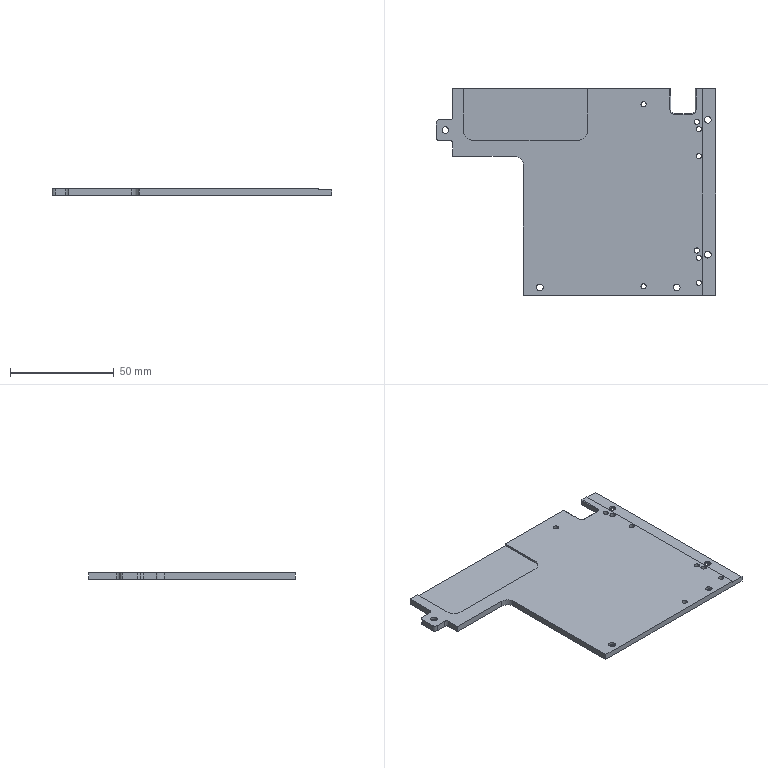CAM job | Mastercam | mm | 16 operations | part box 134.7 x 99.55 x 3
1. Contour (Ramp) | 8 - 8C
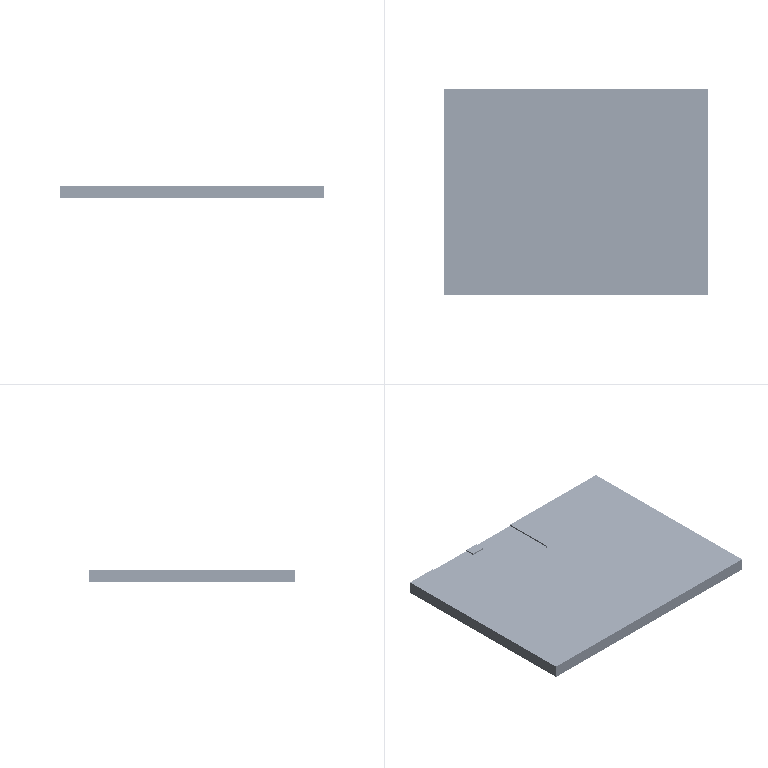2. Contour (Ramp) | 8 - 8C
3. Contour (2D) | 9 - 8J
4. Contour (2D) | 9 - 8J
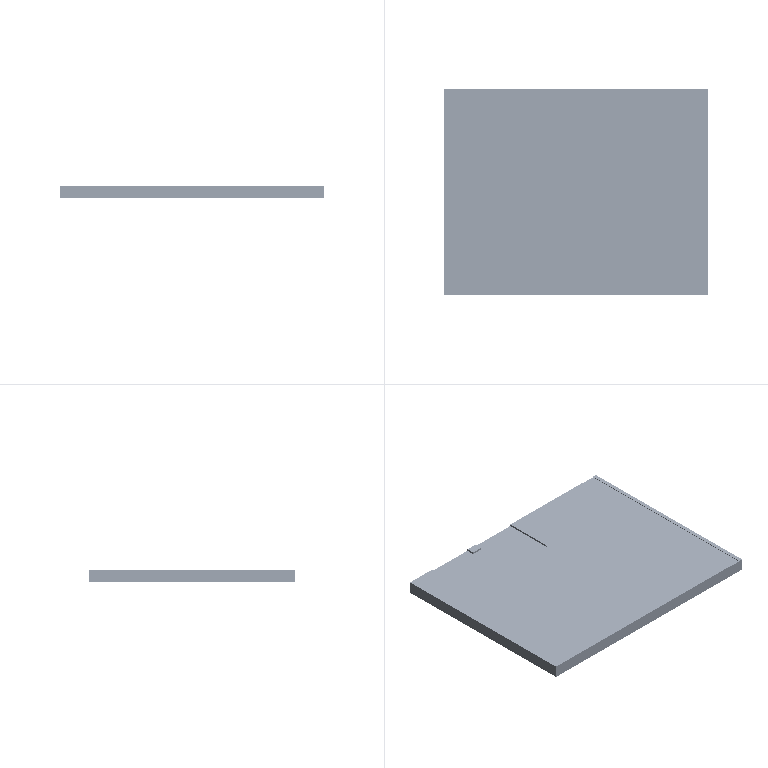5. Contour (2D) | 9 - 8J
6. Drill/Counterbore | 1 - 6 倒角刀
7. Drill/Counterbore | 1 - 6 倒角刀
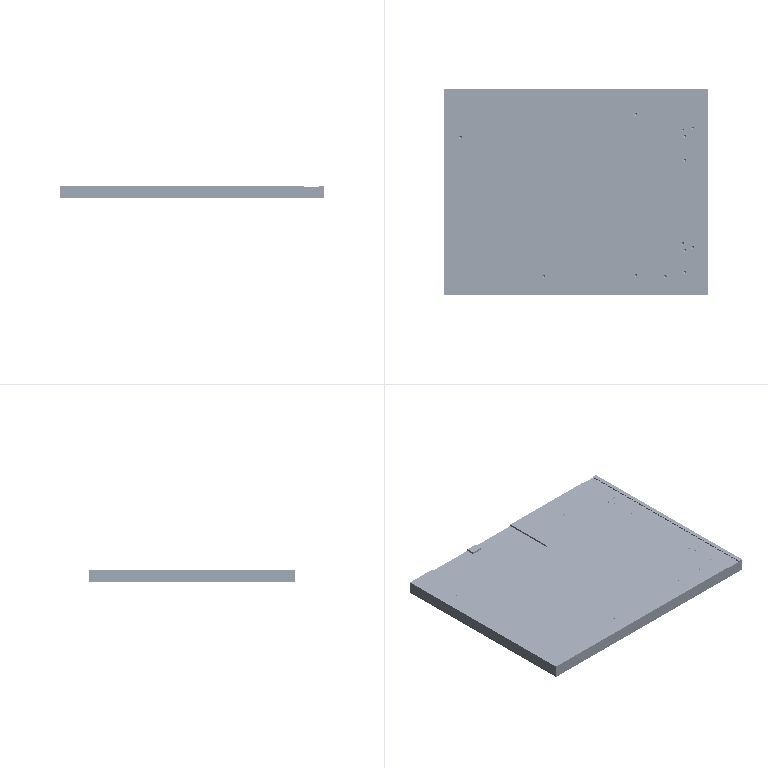8. Peck Drill | 21 - 3.2 钻头
9. Peck Drill | 14 - 2.5 钻头
10. Contour (Ramp) | 8 - 8C
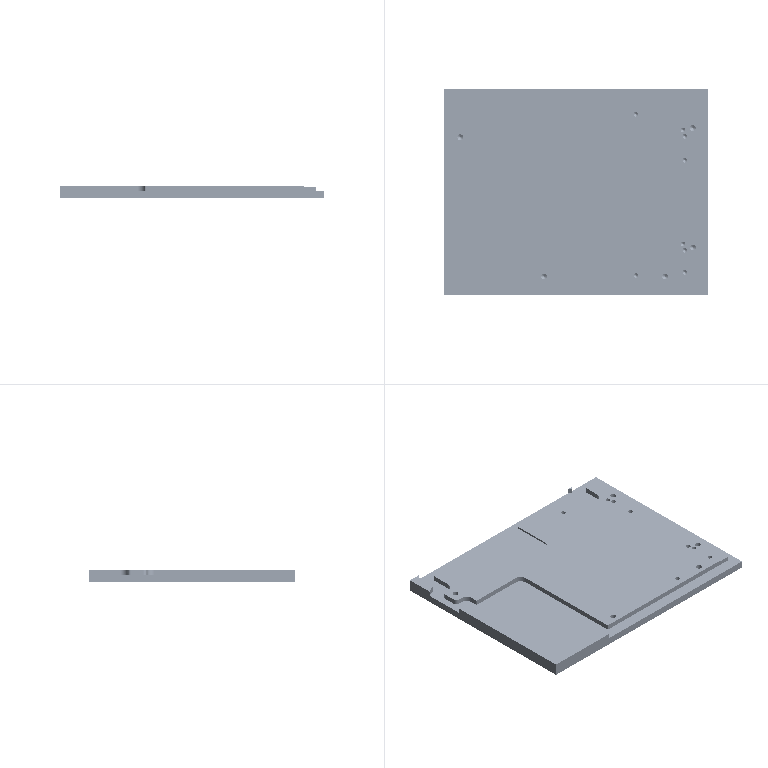11. Contour (2D) | 9 - 8J
12. Contour (Remachining) | 13 - 3J
13. Chamfer Drill | 1 - 6 倒角刀
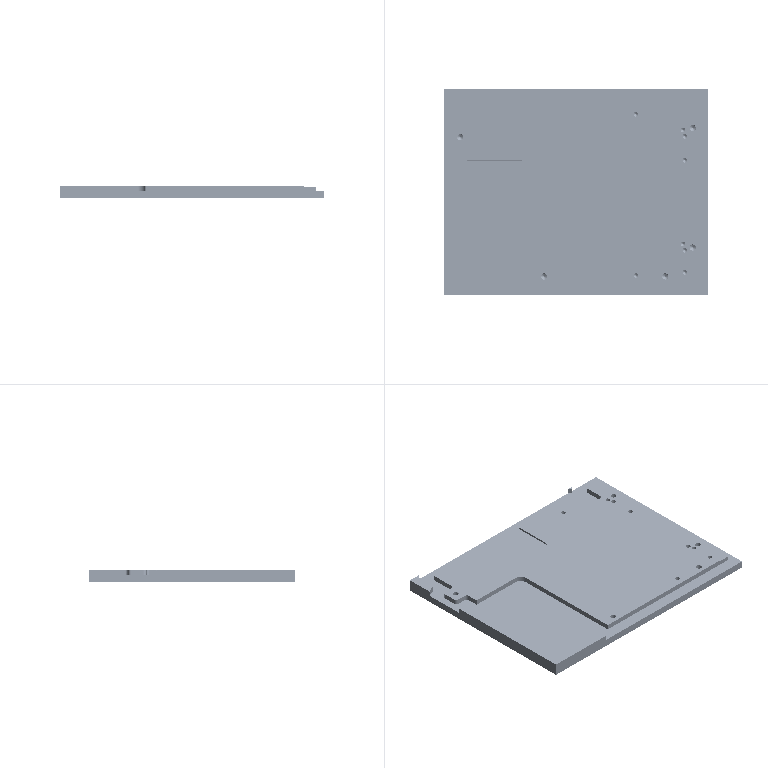14. Chamfer Drill | 1 - 6 倒角刀
15. Contour (2D chamfer) | 1 - 6 倒角刀
16. Model Chamfer | 1 - 6 倒角刀